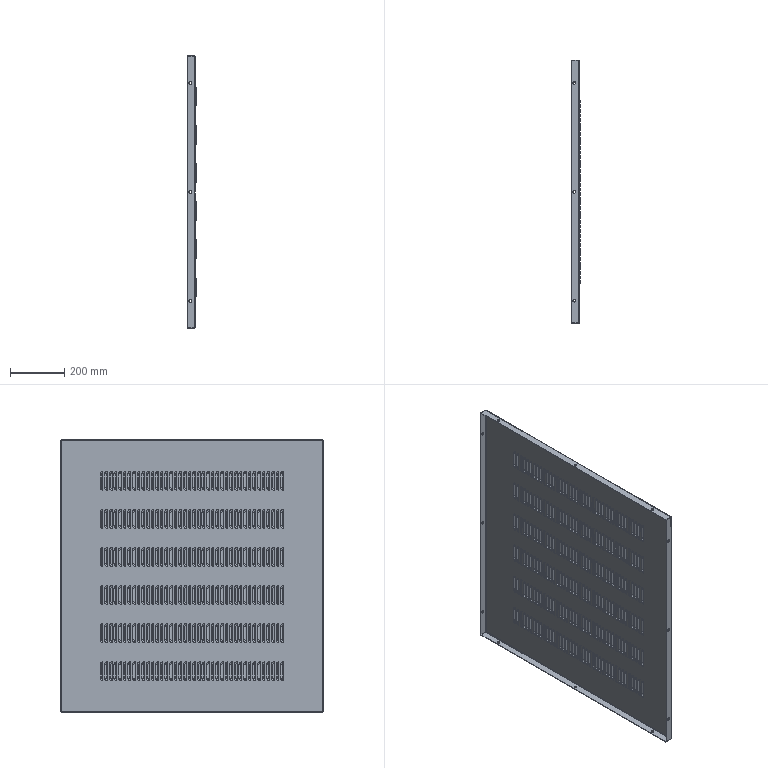Component | SolidWorks | 38SidePlate-2 | 1 solid | 2462 faces | volume 2223173 mm3 | plane 982 | torus 960 | cylinder 512 | spline 8 | commonest cylinder face diameters 10 x264 14 x240 2 x4 6 x4